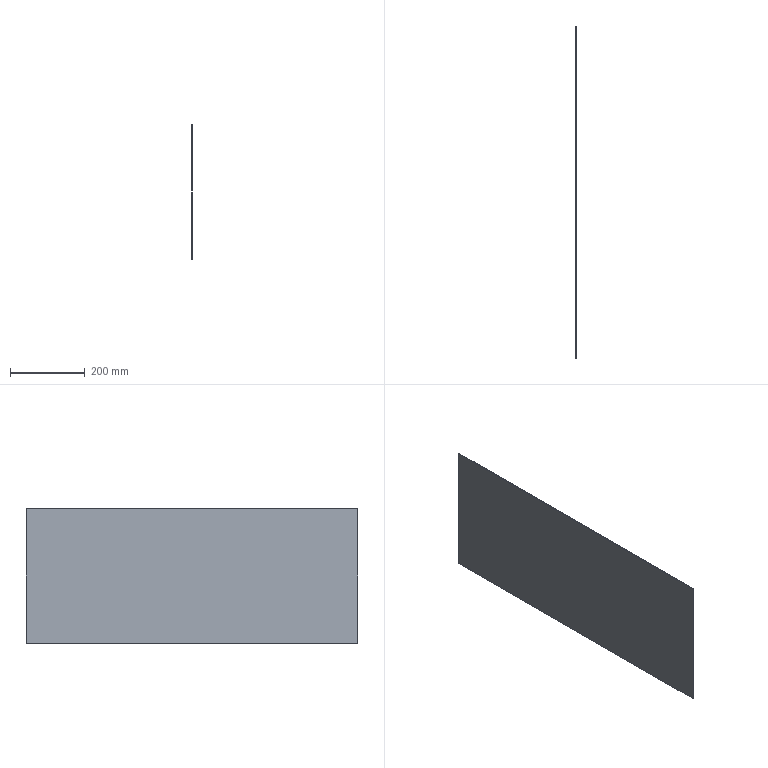Component | NX | COVER_PLATE | 1 solid | 6 faces | box 2 x 889.3 x 360 mm | volume 640298 mm3 | plane 6
STEP:
#1=CARTESIAN_POINT('',(0.,0.,0.));
#2=DIRECTION('',(0.,0.,1.));
#3=DIRECTION('',(1.,0.,0.));
#4=AXIS2_PLACEMENT_3D('',#1,#2,#3);
#5=CARTESIAN_POINT('',(346.,444.651,-606.582));
#6=VERTEX_POINT('',#5);
#7=CARTESIAN_POINT('',(346.,444.651,-246.582));
#8=VERTEX_POINT('',#7);
#9=CARTESIAN_POINT('',(346.,444.651,-700.));
#10=DIRECTION('',(0.,-0.,1.));
#11=VECTOR('',#10,1.);
#12=LINE('',#9,#11);
#13=CARTESIAN_POINT('',(296.926,444.651,216.709));
#14=DIRECTION('',(0.,-1.,-0.));
#15=DIRECTION('',(0.,0.,-1.));
#16=AXIS2_PLACEMENT_3D('',#13,#14,#15);
#17=PLANE('',#16);
#18=CARTESIAN_POINT('',(916.709,49.074));
#19=DIRECTION('',(-1.,0.));
#20=VECTOR('',#19,1.);
#21=LINE('',#18,#20);
#22=(GEOMETRIC_REPRESENTATION_CONTEXT(2)PARAMETRIC_REPRESENTATION_CONTEXT()REPRESENTATION_CONTEXT('',''));
#23=DEFINITIONAL_REPRESENTATION('',(#21),#22);
#24=PCURVE('',#17,#23);
#25=CARTESIAN_POINT('',(346.,-500.,-700.));
#26=DIRECTION('',(-1.,0.,0.));
#27=DIRECTION('',(0.,0.,1.));
#28=AXIS2_PLACEMENT_3D('',#25,#26,#27);
#29=PLANE('',#28);
#30=CARTESIAN_POINT('',(0.,944.651));
#31=DIRECTION('',(1.,-0.));
#32=VECTOR('',#31,1.);
#33=LINE('',#30,#32);
#34=(GEOMETRIC_REPRESENTATION_CONTEXT(2)PARAMETRIC_REPRESENTATION_CONTEXT()REPRESENTATION_CONTEXT('',''));
#35=DEFINITIONAL_REPRESENTATION('',(#33),#34);
#36=PCURVE('',#29,#35);
#37=SURFACE_CURVE('',#12,(#24,#36),.PCURVE_S1.);
#38=EDGE_CURVE('',#6,#8,#37,.T.);
#39=ORIENTED_EDGE('',*,*,#38,.F.);
#40=CARTESIAN_POINT('',(344.,444.651,-606.582));
#41=VERTEX_POINT('',#40);
#42=CARTESIAN_POINT('',(296.926,444.651,-606.582));
#43=DIRECTION('',(-1.,0.,0.));
#44=VECTOR('',#43,1.);
#45=LINE('',#42,#44);
#46=CARTESIAN_POINT('',(823.291,0.));
#47=DIRECTION('',(0.,-1.));
#48=VECTOR('',#47,1.);
#49=LINE('',#46,#48);
#50=(GEOMETRIC_REPRESENTATION_CONTEXT(2)PARAMETRIC_REPRESENTATION_CONTEXT()REPRESENTATION_CONTEXT('',''));
#51=DEFINITIONAL_REPRESENTATION('',(#49),#50);
#52=PCURVE('',#17,#51);
#53=CARTESIAN_POINT('',(345.,0.,-606.582));
#54=DIRECTION('',(0.,0.,1.));
#55=DIRECTION('',(1.,0.,0.));
#56=AXIS2_PLACEMENT_3D('',#53,#54,#55);
#57=PLANE('',#56);
#58=CARTESIAN_POINT('',(-48.074,444.651));
#59=DIRECTION('',(-1.,0.));
#60=VECTOR('',#59,1.);
#61=LINE('',#58,#60);
#62=(GEOMETRIC_REPRESENTATION_CONTEXT(2)PARAMETRIC_REPRESENTATION_CONTEXT()REPRESENTATION_CONTEXT('',''));
#63=DEFINITIONAL_REPRESENTATION('',(#61),#62);
#64=PCURVE('',#57,#63);
#65=SURFACE_CURVE('',#45,(#52,#64),.PCURVE_S1.);
#66=EDGE_CURVE('',#6,#41,#65,.T.);
#67=ORIENTED_EDGE('',*,*,#66,.T.);
#68=CARTESIAN_POINT('',(344.,444.651,-246.582));
#69=VERTEX_POINT('',#68);
#70=CARTESIAN_POINT('',(344.,444.651,-700.));
#71=DIRECTION('',(0.,-0.,1.));
#72=VECTOR('',#71,1.);
#73=LINE('',#70,#72);
#74=CARTESIAN_POINT('',(916.709,47.074));
#75=DIRECTION('',(-1.,0.));
#76=VECTOR('',#75,1.);
#77=LINE('',#74,#76);
#78=(GEOMETRIC_REPRESENTATION_CONTEXT(2)PARAMETRIC_REPRESENTATION_CONTEXT()REPRESENTATION_CONTEXT('',''));
#79=DEFINITIONAL_REPRESENTATION('',(#77),#78);
#80=PCURVE('',#17,#79);
#81=CARTESIAN_POINT('',(344.,-500.,-700.));
#82=DIRECTION('',(-1.,0.,0.));
#83=DIRECTION('',(0.,0.,1.));
#84=AXIS2_PLACEMENT_3D('',#81,#82,#83);
#85=PLANE('',#84);
#86=CARTESIAN_POINT('',(0.,944.651));
#87=DIRECTION('',(1.,-0.));
#88=VECTOR('',#87,1.);
#89=LINE('',#86,#88);
#90=(GEOMETRIC_REPRESENTATION_CONTEXT(2)PARAMETRIC_REPRESENTATION_CONTEXT()REPRESENTATION_CONTEXT('',''));
#91=DEFINITIONAL_REPRESENTATION('',(#89),#90);
#92=PCURVE('',#85,#91);
#93=SURFACE_CURVE('',#73,(#80,#92),.PCURVE_S1.);
#94=EDGE_CURVE('',#41,#69,#93,.T.);
#95=ORIENTED_EDGE('',*,*,#94,.T.);
#96=CARTESIAN_POINT('',(370.,444.651,-246.582));
#97=DIRECTION('',(1.,0.,0.));
#98=VECTOR('',#97,1.);
#99=LINE('',#96,#98);
#100=CARTESIAN_POINT('',(463.291,73.074));
#101=DIRECTION('',(0.,1.));
#102=VECTOR('',#101,1.);
#103=LINE('',#100,#102);
#104=(GEOMETRIC_REPRESENTATION_CONTEXT(2)PARAMETRIC_REPRESENTATION_CONTEXT()REPRESENTATION_CONTEXT('',''));
#105=DEFINITIONAL_REPRESENTATION('',(#103),#104);
#106=PCURVE('',#17,#105);
#107=CARTESIAN_POINT('',(370.,444.651,-246.582));
#108=DIRECTION('',(0.,0.,-1.));
#109=DIRECTION('',(-1.,0.,0.));
#110=AXIS2_PLACEMENT_3D('',#107,#108,#109);
#111=PLANE('',#110);
#112=CARTESIAN_POINT('',(0.,0.));
#113=DIRECTION('',(-1.,0.));
#114=VECTOR('',#113,1.);
#115=LINE('',#112,#114);
#116=(GEOMETRIC_REPRESENTATION_CONTEXT(2)PARAMETRIC_REPRESENTATION_CONTEXT()REPRESENTATION_CONTEXT('',''));
#117=DEFINITIONAL_REPRESENTATION('',(#115),#116);
#118=PCURVE('',#111,#117);
#119=SURFACE_CURVE('',#99,(#106,#118),.PCURVE_S1.);
#120=EDGE_CURVE('',#69,#8,#119,.T.);
#121=ORIENTED_EDGE('',*,*,#120,.T.);
#122=EDGE_LOOP('',(#39,#67,#95,#121));
#123=FACE_BOUND('',#122,.T.);
#124=ADVANCED_FACE('',(#123),#17,.F.);
#125=CARTESIAN_POINT('',(344.,-444.651,-246.582));
#126=VERTEX_POINT('',#125);
#127=CARTESIAN_POINT('',(344.,-444.651,-606.582));
#128=VERTEX_POINT('',#127);
#129=CARTESIAN_POINT('',(344.,-444.651,-700.));
#130=DIRECTION('',(0.,0.,-1.));
#131=VECTOR('',#130,1.);
#132=LINE('',#129,#131);
#133=CARTESIAN_POINT('',(5.,-444.651,226.709));
#134=DIRECTION('',(0.,1.,0.));
#135=DIRECTION('',(0.,0.,1.));
#136=AXIS2_PLACEMENT_3D('',#133,#134,#135);
#137=PLANE('',#136);
#138=CARTESIAN_POINT('',(-926.709,339.));
#139=DIRECTION('',(-1.,0.));
#140=VECTOR('',#139,1.);
#141=LINE('',#138,#140);
#142=(GEOMETRIC_REPRESENTATION_CONTEXT(2)PARAMETRIC_REPRESENTATION_CONTEXT()REPRESENTATION_CONTEXT('',''));
#143=DEFINITIONAL_REPRESENTATION('',(#141),#142);
#144=PCURVE('',#137,#143);
#145=CARTESIAN_POINT('',(0.,55.349));
#146=DIRECTION('',(-1.,0.));
#147=VECTOR('',#146,1.);
#148=LINE('',#145,#147);
#149=(GEOMETRIC_REPRESENTATION_CONTEXT(2)PARAMETRIC_REPRESENTATION_CONTEXT()REPRESENTATION_CONTEXT('',''));
#150=DEFINITIONAL_REPRESENTATION('',(#148),#149);
#151=PCURVE('',#85,#150);
#152=SURFACE_CURVE('',#132,(#144,#151),.PCURVE_S1.);
#153=EDGE_CURVE('',#126,#128,#152,.T.);
#154=ORIENTED_EDGE('',*,*,#153,.T.);
#155=CARTESIAN_POINT('',(346.,-444.651,-606.582));
#156=VERTEX_POINT('',#155);
#157=CARTESIAN_POINT('',(5.,-444.651,-606.582));
#158=DIRECTION('',(1.,0.,0.));
#159=VECTOR('',#158,1.);
#160=LINE('',#157,#159);
#161=CARTESIAN_POINT('',(-833.291,0.));
#162=DIRECTION('',(0.,1.));
#163=VECTOR('',#162,1.);
#164=LINE('',#161,#163);
#165=(GEOMETRIC_REPRESENTATION_CONTEXT(2)PARAMETRIC_REPRESENTATION_CONTEXT()REPRESENTATION_CONTEXT('',''));
#166=DEFINITIONAL_REPRESENTATION('',(#164),#165);
#167=PCURVE('',#137,#166);
#168=CARTESIAN_POINT('',(-340.,-444.651));
#169=DIRECTION('',(1.,0.));
#170=VECTOR('',#169,1.);
#171=LINE('',#168,#170);
#172=(GEOMETRIC_REPRESENTATION_CONTEXT(2)PARAMETRIC_REPRESENTATION_CONTEXT()REPRESENTATION_CONTEXT('',''));
#173=DEFINITIONAL_REPRESENTATION('',(#171),#172);
#174=PCURVE('',#57,#173);
#175=SURFACE_CURVE('',#160,(#167,#174),.PCURVE_S1.);
#176=EDGE_CURVE('',#128,#156,#175,.T.);
#177=ORIENTED_EDGE('',*,*,#176,.T.);
#178=CARTESIAN_POINT('',(346.,-444.651,-246.582));
#179=VERTEX_POINT('',#178);
#180=CARTESIAN_POINT('',(346.,-444.651,-700.));
#181=DIRECTION('',(0.,0.,-1.));
#182=VECTOR('',#181,1.);
#183=LINE('',#180,#182);
#184=CARTESIAN_POINT('',(-926.709,341.));
#185=DIRECTION('',(-1.,0.));
#186=VECTOR('',#185,1.);
#187=LINE('',#184,#186);
#188=(GEOMETRIC_REPRESENTATION_CONTEXT(2)PARAMETRIC_REPRESENTATION_CONTEXT()REPRESENTATION_CONTEXT('',''));
#189=DEFINITIONAL_REPRESENTATION('',(#187),#188);
#190=PCURVE('',#137,#189);
#191=CARTESIAN_POINT('',(0.,55.349));
#192=DIRECTION('',(-1.,0.));
#193=VECTOR('',#192,1.);
#194=LINE('',#191,#193);
#195=(GEOMETRIC_REPRESENTATION_CONTEXT(2)PARAMETRIC_REPRESENTATION_CONTEXT()REPRESENTATION_CONTEXT('',''));
#196=DEFINITIONAL_REPRESENTATION('',(#194),#195);
#197=PCURVE('',#29,#196);
#198=SURFACE_CURVE('',#183,(#190,#197),.PCURVE_S1.);
#199=EDGE_CURVE('',#179,#156,#198,.T.);
#200=ORIENTED_EDGE('',*,*,#199,.F.);
#201=CARTESIAN_POINT('',(370.,-444.651,-246.582));
#202=DIRECTION('',(1.,0.,0.));
#203=VECTOR('',#202,1.);
#204=LINE('',#201,#203);
#205=CARTESIAN_POINT('',(-473.291,365.));
#206=DIRECTION('',(0.,1.));
#207=VECTOR('',#206,1.);
#208=LINE('',#205,#207);
#209=(GEOMETRIC_REPRESENTATION_CONTEXT(2)PARAMETRIC_REPRESENTATION_CONTEXT()REPRESENTATION_CONTEXT('',''));
#210=DEFINITIONAL_REPRESENTATION('',(#208),#209);
#211=PCURVE('',#137,#210);
#212=CARTESIAN_POINT('',(0.,-889.302));
#213=DIRECTION('',(-1.,0.));
#214=VECTOR('',#213,1.);
#215=LINE('',#212,#214);
#216=(GEOMETRIC_REPRESENTATION_CONTEXT(2)PARAMETRIC_REPRESENTATION_CONTEXT()REPRESENTATION_CONTEXT('',''));
#217=DEFINITIONAL_REPRESENTATION('',(#215),#216);
#218=PCURVE('',#111,#217);
#219=SURFACE_CURVE('',#204,(#211,#218),.PCURVE_S1.);
#220=EDGE_CURVE('',#126,#179,#219,.T.);
#221=ORIENTED_EDGE('',*,*,#220,.F.);
#222=EDGE_LOOP('',(#154,#177,#200,#221));
#223=FACE_BOUND('',#222,.T.);
#224=ADVANCED_FACE('',(#223),#137,.F.);
#225=ORIENTED_EDGE('',*,*,#120,.F.);
#226=CARTESIAN_POINT('',(344.,-500.,-246.582));
#227=DIRECTION('',(0.,-1.,0.));
#228=VECTOR('',#227,1.);
#229=LINE('',#226,#228);
#230=CARTESIAN_POINT('',(26.,-944.651));
#231=DIRECTION('',(0.,-1.));
#232=VECTOR('',#231,1.);
#233=LINE('',#230,#232);
#234=(GEOMETRIC_REPRESENTATION_CONTEXT(2)PARAMETRIC_REPRESENTATION_CONTEXT()REPRESENTATION_CONTEXT('',''));
#235=DEFINITIONAL_REPRESENTATION('',(#233),#234);
#236=PCURVE('',#111,#235);
#237=CARTESIAN_POINT('',(453.418,0.));
#238=DIRECTION('',(0.,-1.));
#239=VECTOR('',#238,1.);
#240=LINE('',#237,#239);
#241=(GEOMETRIC_REPRESENTATION_CONTEXT(2)PARAMETRIC_REPRESENTATION_CONTEXT()REPRESENTATION_CONTEXT('',''));
#242=DEFINITIONAL_REPRESENTATION('',(#240),#241);
#243=PCURVE('',#85,#242);
#244=SURFACE_CURVE('',#229,(#236,#243),.PCURVE_S1.);
#245=EDGE_CURVE('',#69,#126,#244,.T.);
#246=ORIENTED_EDGE('',*,*,#245,.T.);
#247=ORIENTED_EDGE('',*,*,#220,.T.);
#248=CARTESIAN_POINT('',(346.,-500.,-246.582));
#249=DIRECTION('',(0.,-1.,0.));
#250=VECTOR('',#249,1.);
#251=LINE('',#248,#250);
#252=CARTESIAN_POINT('',(24.,-944.651));
#253=DIRECTION('',(0.,-1.));
#254=VECTOR('',#253,1.);
#255=LINE('',#252,#254);
#256=(GEOMETRIC_REPRESENTATION_CONTEXT(2)PARAMETRIC_REPRESENTATION_CONTEXT()REPRESENTATION_CONTEXT('',''));
#257=DEFINITIONAL_REPRESENTATION('',(#255),#256);
#258=PCURVE('',#111,#257);
#259=CARTESIAN_POINT('',(453.418,0.));
#260=DIRECTION('',(0.,-1.));
#261=VECTOR('',#260,1.);
#262=LINE('',#259,#261);
#263=(GEOMETRIC_REPRESENTATION_CONTEXT(2)PARAMETRIC_REPRESENTATION_CONTEXT()REPRESENTATION_CONTEXT('',''));
#264=DEFINITIONAL_REPRESENTATION('',(#262),#263);
#265=PCURVE('',#29,#264);
#266=SURFACE_CURVE('',#251,(#258,#265),.PCURVE_S1.);
#267=EDGE_CURVE('',#8,#179,#266,.T.);
#268=ORIENTED_EDGE('',*,*,#267,.F.);
#269=EDGE_LOOP('',(#225,#246,#247,#268));
#270=FACE_BOUND('',#269,.T.);
#271=ADVANCED_FACE('',(#270),#111,.F.);
#272=CARTESIAN_POINT('',(344.,-500.,-606.582));
#273=DIRECTION('',(0.,-1.,0.));
#274=VECTOR('',#273,1.);
#275=LINE('',#272,#274);
#276=CARTESIAN_POINT('',(93.418,0.));
#277=DIRECTION('',(0.,-1.));
#278=VECTOR('',#277,1.);
#279=LINE('',#276,#278);
#280=(GEOMETRIC_REPRESENTATION_CONTEXT(2)PARAMETRIC_REPRESENTATION_CONTEXT()REPRESENTATION_CONTEXT('',''));
#281=DEFINITIONAL_REPRESENTATION('',(#279),#280);
#282=PCURVE('',#85,#281);
#283=CARTESIAN_POINT('',(-1.,-500.));
#284=DIRECTION('',(0.,-1.));
#285=VECTOR('',#284,1.);
#286=LINE('',#283,#285);
#287=(GEOMETRIC_REPRESENTATION_CONTEXT(2)PARAMETRIC_REPRESENTATION_CONTEXT()REPRESENTATION_CONTEXT('',''));
#288=DEFINITIONAL_REPRESENTATION('',(#286),#287);
#289=PCURVE('',#57,#288);
#290=SURFACE_CURVE('',#275,(#282,#289),.PCURVE_S1.);
#291=EDGE_CURVE('',#41,#128,#290,.T.);
#292=ORIENTED_EDGE('',*,*,#291,.T.);
#293=ORIENTED_EDGE('',*,*,#153,.F.);
#294=ORIENTED_EDGE('',*,*,#245,.F.);
#295=ORIENTED_EDGE('',*,*,#94,.F.);
#296=EDGE_LOOP('',(#292,#293,#294,#295));
#297=FACE_BOUND('',#296,.T.);
#298=ADVANCED_FACE('',(#297),#85,.T.);
#299=ORIENTED_EDGE('',*,*,#199,.T.);
#300=CARTESIAN_POINT('',(346.,-500.,-606.582));
#301=DIRECTION('',(0.,-1.,0.));
#302=VECTOR('',#301,1.);
#303=LINE('',#300,#302);
#304=CARTESIAN_POINT('',(93.418,0.));
#305=DIRECTION('',(0.,-1.));
#306=VECTOR('',#305,1.);
#307=LINE('',#304,#306);
#308=(GEOMETRIC_REPRESENTATION_CONTEXT(2)PARAMETRIC_REPRESENTATION_CONTEXT()REPRESENTATION_CONTEXT('',''));
#309=DEFINITIONAL_REPRESENTATION('',(#307),#308);
#310=PCURVE('',#29,#309);
#311=CARTESIAN_POINT('',(1.,-500.));
#312=DIRECTION('',(0.,-1.));
#313=VECTOR('',#312,1.);
#314=LINE('',#311,#313);
#315=(GEOMETRIC_REPRESENTATION_CONTEXT(2)PARAMETRIC_REPRESENTATION_CONTEXT()REPRESENTATION_CONTEXT('',''));
#316=DEFINITIONAL_REPRESENTATION('',(#314),#315);
#317=PCURVE('',#57,#316);
#318=SURFACE_CURVE('',#303,(#310,#317),.PCURVE_S1.);
#319=EDGE_CURVE('',#6,#156,#318,.T.);
#320=ORIENTED_EDGE('',*,*,#319,.F.);
#321=ORIENTED_EDGE('',*,*,#38,.T.);
#322=ORIENTED_EDGE('',*,*,#267,.T.);
#323=EDGE_LOOP('',(#299,#320,#321,#322));
#324=FACE_BOUND('',#323,.T.);
#325=ADVANCED_FACE('',(#324),#29,.F.);
#326=ORIENTED_EDGE('',*,*,#291,.F.);
#327=ORIENTED_EDGE('',*,*,#66,.F.);
#328=ORIENTED_EDGE('',*,*,#319,.T.);
#329=ORIENTED_EDGE('',*,*,#176,.F.);
#330=EDGE_LOOP('',(#326,#327,#328,#329));
#331=FACE_BOUND('',#330,.T.);
#332=ADVANCED_FACE('',(#331),#57,.F.);
#333=CLOSED_SHELL('',(#124,#224,#271,#298,#325,#332));
#334=MANIFOLD_SOLID_BREP('',#333);
#335=(LENGTH_UNIT()NAMED_UNIT(*)SI_UNIT(.MILLI.,.METRE.));
#336=UNCERTAINTY_MEASURE_WITH_UNIT(LENGTH_MEASURE(0.0000001),#335,'','');
#337=(NAMED_UNIT(*)PLANE_ANGLE_UNIT()SI_UNIT($,.RADIAN.));
#338=(NAMED_UNIT(*)SI_UNIT($,.STERADIAN.)SOLID_ANGLE_UNIT());
#339=(GEOMETRIC_REPRESENTATION_CONTEXT(3)GLOBAL_UNCERTAINTY_ASSIGNED_CONTEXT((#336))GLOBAL_UNIT_ASSIGNED_CONTEXT((#335,#337,#338))REPRESENTATION_CONTEXT('',''));
#340=ADVANCED_BREP_SHAPE_REPRESENTATION('',(#4,#334),#339);